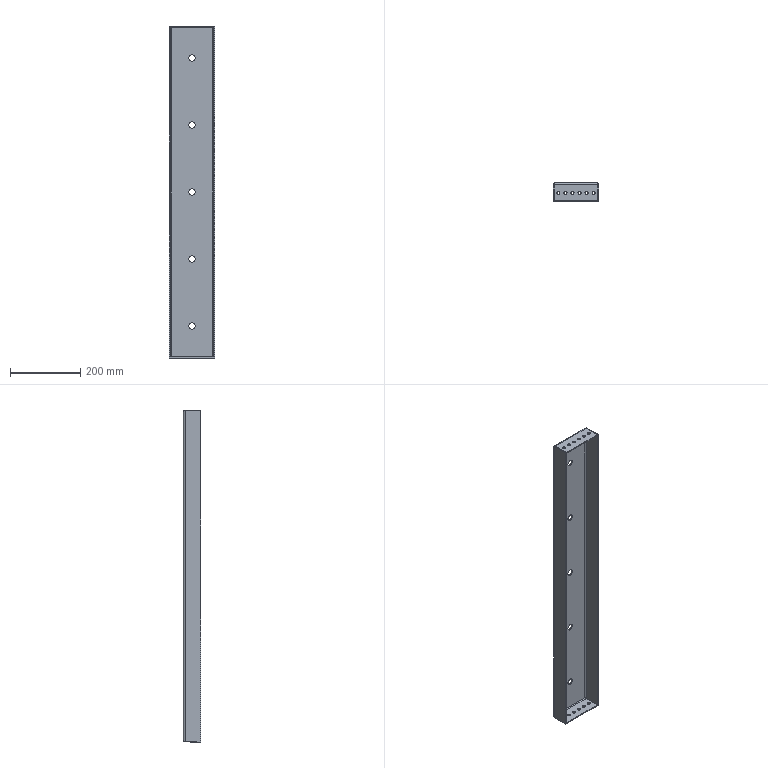Component | SolidWorks | CapacitorBeamF6-2 | 1 solid | 72 faces | volume 650710 mm3 | cylinder 42 | plane 22 | spline 8 | commonest cylinder face diameters 9 x24 18 x10 5 x4 11 x4